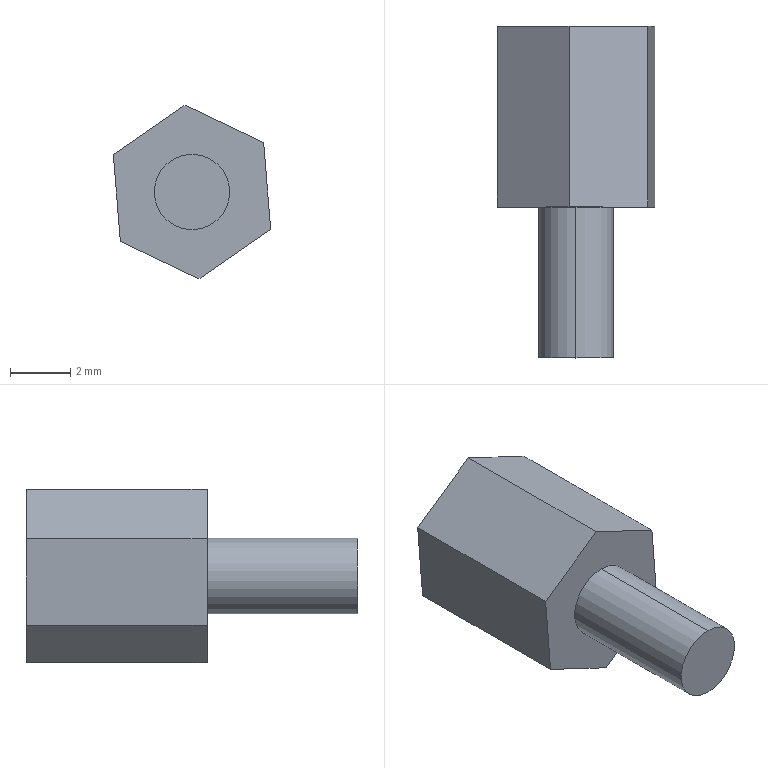Component | SolidWorks | Bolt-11 | 1 solid | 14 faces | box 5.22 x 11 x 5.75 mm | volume 130 mm3 | plane 10 | cylinder 4 | commonest cylinder face diameters 2.5 x4
build123d program:
from build123d import *

# Parameters (mm, degrees)
BOSS_EXTRUDE1_DEPTH = 6
SKETCH2_R           = 1.25
CUT_EXTRUDE1_DEPTH  = 5
SKETCH3_R           = 1.25
BOSS_EXTRUDE2_DEPTH = 5


with BuildPart() as part:
    # Sketch1 → Boss-Extrude1 (new body)
    with BuildSketch(Plane.XY):
        Polygon((2.877, 0.2318), (1.238, 2.608), (-1.639, 2.376), (-2.877, -0.2318), (-1.238, -2.608), (1.639, -2.376), align=None)
    extrude(amount=BOSS_EXTRUDE1_DEPTH)

    # Sketch2 → Cut-Extrude1 (cut)
    with BuildSketch(Plane(origin=(0, 0, 0), x_dir=(-1, 0, 0), z_dir=(0, 0, -1))):
        Circle(SKETCH2_R)
    extrude(amount=-CUT_EXTRUDE1_DEPTH, mode=Mode.SUBTRACT)

    # Sketch3 → Boss-Extrude2 (add)
    with BuildSketch(Plane.XY.offset(6)):
        with Locations(Location((0, 0, 0), (0, 0, 180))):
            Circle(SKETCH3_R)
    extrude(amount=BOSS_EXTRUDE2_DEPTH)


solid = part.part

# Placed as in the assembly
solid = solid.moved(Location((27.326, 19.961, 70.581), (90, 0, 90)))
STEP:
#1=COLOUR_RGB('',0.7922,0.8196,0.9333);
#2=FILL_AREA_STYLE_COLOUR('',#1);
#3=FILL_AREA_STYLE('',(#2));
#4=SURFACE_STYLE_FILL_AREA(#3);
#5=SURFACE_SIDE_STYLE('',(#4));
#6=SURFACE_STYLE_USAGE(.BOTH.,#5);
#7=PRESENTATION_STYLE_ASSIGNMENT((#6));
#8=CARTESIAN_POINT('',(1.076,0.3528,2.73));
#9=VERTEX_POINT('',#8);
#10=CARTESIAN_POINT('',(1.076,0.3528,2.828));
#11=VERTEX_POINT('',#10);
#12=CARTESIAN_POINT('',(1.076,0.3528,2.779));
#13=DIRECTION('',(-0.,-1.,-0.));
#14=DIRECTION('',(0.,0.,-1.));
#15=AXIS2_PLACEMENT_3D('',#12,#13,#14);
#16=CIRCLE('',#15,0.04921);
#17=EDGE_CURVE('',#9,#11,#16,.T.);
#18=ORIENTED_EDGE('',*,*,#17,.F.);
#19=CARTESIAN_POINT('',(1.076,0.5496,2.73));
#20=VERTEX_POINT('',#19);
#21=CARTESIAN_POINT('',(1.076,0.3528,2.73));
#22=DIRECTION('',(0.,1.,0.));
#23=VECTOR('',#22,39.37);
#24=LINE('',#21,#23);
#25=EDGE_CURVE('',#9,#20,#24,.T.);
#26=ORIENTED_EDGE('',*,*,#25,.T.);
#27=CARTESIAN_POINT('',(1.076,0.5496,2.828));
#28=VERTEX_POINT('',#27);
#29=CARTESIAN_POINT('',(1.076,0.5496,2.779));
#30=DIRECTION('',(-0.,-1.,-0.));
#31=DIRECTION('',(0.,0.,-1.));
#32=AXIS2_PLACEMENT_3D('',#29,#30,#31);
#33=CIRCLE('',#32,0.04921);
#34=EDGE_CURVE('',#20,#28,#33,.T.);
#35=ORIENTED_EDGE('',*,*,#34,.T.);
#36=CARTESIAN_POINT('',(1.076,0.3528,2.828));
#37=DIRECTION('',(0.,1.,0.));
#38=VECTOR('',#37,39.37);
#39=LINE('',#36,#38);
#40=EDGE_CURVE('',#11,#28,#39,.T.);
#41=ORIENTED_EDGE('',*,*,#40,.F.);
#42=EDGE_LOOP('',(#18,#26,#35,#41));
#43=FACE_OUTER_BOUND('',#42,.T.);
#44=CARTESIAN_POINT('',(1.076,0.3528,2.779));
#45=DIRECTION('',(0.,1.,0.));
#46=DIRECTION('',(-0.,-0.,1.));
#47=AXIS2_PLACEMENT_3D('',#44,#45,#46);
#48=CYLINDRICAL_SURFACE('',#47,0.04921);
#49=ADVANCED_FACE('',(#43),#48,.T.);
#50=CARTESIAN_POINT('',(1.076,0.589,2.73));
#51=VERTEX_POINT('',#50);
#52=CARTESIAN_POINT('',(1.076,0.589,2.828));
#53=VERTEX_POINT('',#52);
#54=CARTESIAN_POINT('',(1.076,0.589,2.779));
#55=DIRECTION('',(0.,1.,0.));
#56=DIRECTION('',(-0.,-0.,1.));
#57=AXIS2_PLACEMENT_3D('',#54,#55,#56);
#58=CIRCLE('',#57,0.04921);
#59=EDGE_CURVE('',#51,#53,#58,.T.);
#60=ORIENTED_EDGE('',*,*,#59,.F.);
#61=CARTESIAN_POINT('',(1.076,0.7859,2.73));
#62=VERTEX_POINT('',#61);
#63=CARTESIAN_POINT('',(1.076,0.589,2.73));
#64=DIRECTION('',(0.,1.,0.));
#65=VECTOR('',#64,39.37);
#66=LINE('',#63,#65);
#67=EDGE_CURVE('',#51,#62,#66,.T.);
#68=ORIENTED_EDGE('',*,*,#67,.T.);
#69=CARTESIAN_POINT('',(1.076,0.7859,2.828));
#70=VERTEX_POINT('',#69);
#71=CARTESIAN_POINT('',(1.076,0.7859,2.779));
#72=DIRECTION('',(0.,1.,0.));
#73=DIRECTION('',(-0.,-0.,1.));
#74=AXIS2_PLACEMENT_3D('',#71,#72,#73);
#75=CIRCLE('',#74,0.04921);
#76=EDGE_CURVE('',#62,#70,#75,.T.);
#77=ORIENTED_EDGE('',*,*,#76,.T.);
#78=CARTESIAN_POINT('',(1.076,0.589,2.828));
#79=DIRECTION('',(0.,1.,0.));
#80=VECTOR('',#79,39.37);
#81=LINE('',#78,#80);
#82=EDGE_CURVE('',#53,#70,#81,.T.);
#83=ORIENTED_EDGE('',*,*,#82,.F.);
#84=EDGE_LOOP('',(#60,#68,#77,#83));
#85=FACE_OUTER_BOUND('',#84,.T.);
#86=CARTESIAN_POINT('',(1.076,0.589,2.779));
#87=DIRECTION('',(0.,1.,0.));
#88=DIRECTION('',(-0.,-0.,1.));
#89=AXIS2_PLACEMENT_3D('',#86,#87,#88);
#90=CYLINDRICAL_SURFACE('',#89,0.04921);
#91=ADVANCED_FACE('',(#85),#90,.F.);
#92=CARTESIAN_POINT('',(0.9823,0.7859,2.714));
#93=VERTEX_POINT('',#92);
#94=CARTESIAN_POINT('',(1.085,0.7859,2.665));
#95=VERTEX_POINT('',#94);
#96=CARTESIAN_POINT('',(0.9823,0.7859,2.714));
#97=DIRECTION('',(0.9034,-0.,-0.4289));
#98=VECTOR('',#97,39.37);
#99=LINE('',#96,#98);
#100=EDGE_CURVE('',#93,#95,#99,.T.);
#101=ORIENTED_EDGE('',*,*,#100,.T.);
#102=CARTESIAN_POINT('',(1.085,0.5496,2.665));
#103=VERTEX_POINT('',#102);
#104=CARTESIAN_POINT('',(1.085,0.5496,2.665));
#105=DIRECTION('',(0.,1.,0.));
#106=VECTOR('',#105,39.37);
#107=LINE('',#104,#106);
#108=EDGE_CURVE('',#103,#95,#107,.T.);
#109=ORIENTED_EDGE('',*,*,#108,.F.);
#110=CARTESIAN_POINT('',(0.9823,0.5496,2.714));
#111=VERTEX_POINT('',#110);
#112=CARTESIAN_POINT('',(0.9823,0.5496,2.714));
#113=DIRECTION('',(0.9034,-0.,-0.4289));
#114=VECTOR('',#113,39.37);
#115=LINE('',#112,#114);
#116=EDGE_CURVE('',#111,#103,#115,.T.);
#117=ORIENTED_EDGE('',*,*,#116,.F.);
#118=CARTESIAN_POINT('',(0.9823,0.5496,2.714));
#119=DIRECTION('',(0.,1.,0.));
#120=VECTOR('',#119,39.37);
#121=LINE('',#118,#120);
#122=EDGE_CURVE('',#111,#93,#121,.T.);
#123=ORIENTED_EDGE('',*,*,#122,.T.);
#124=EDGE_LOOP('',(#101,#109,#117,#123));
#125=FACE_OUTER_BOUND('',#124,.T.);
#126=CARTESIAN_POINT('',(0.9823,0.5496,2.714));
#127=DIRECTION('',(0.4289,-0.,0.9034));
#128=DIRECTION('',(-0.9034,0.,0.4289));
#129=AXIS2_PLACEMENT_3D('',#126,#127,#128);
#130=PLANE('',#129);
#131=ADVANCED_FACE('',(#125),#130,.F.);
#132=CARTESIAN_POINT('',(1.179,0.7859,2.73));
#133=VERTEX_POINT('',#132);
#134=CARTESIAN_POINT('',(1.085,0.7859,2.665));
#135=DIRECTION('',(0.8231,-0.,0.5679));
#136=VECTOR('',#135,39.37);
#137=LINE('',#134,#136);
#138=EDGE_CURVE('',#95,#133,#137,.T.);
#139=ORIENTED_EDGE('',*,*,#138,.T.);
#140=CARTESIAN_POINT('',(1.179,0.5496,2.73));
#141=VERTEX_POINT('',#140);
#142=CARTESIAN_POINT('',(1.179,0.5496,2.73));
#143=DIRECTION('',(0.,1.,0.));
#144=VECTOR('',#143,39.37);
#145=LINE('',#142,#144);
#146=EDGE_CURVE('',#141,#133,#145,.T.);
#147=ORIENTED_EDGE('',*,*,#146,.F.);
#148=CARTESIAN_POINT('',(1.085,0.5496,2.665));
#149=DIRECTION('',(0.8231,-0.,0.5679));
#150=VECTOR('',#149,39.37);
#151=LINE('',#148,#150);
#152=EDGE_CURVE('',#103,#141,#151,.T.);
#153=ORIENTED_EDGE('',*,*,#152,.F.);
#154=ORIENTED_EDGE('',*,*,#108,.T.);
#155=EDGE_LOOP('',(#139,#147,#153,#154));
#156=FACE_OUTER_BOUND('',#155,.T.);
#157=CARTESIAN_POINT('',(1.085,0.5496,2.665));
#158=DIRECTION('',(-0.5679,-0.,0.8231));
#159=DIRECTION('',(-0.8231,0.,-0.5679));
#160=AXIS2_PLACEMENT_3D('',#157,#158,#159);
#161=PLANE('',#160);
#162=ADVANCED_FACE('',(#156),#161,.F.);
#163=CARTESIAN_POINT('',(1.169,0.7859,2.843));
#164=VERTEX_POINT('',#163);
#165=CARTESIAN_POINT('',(1.179,0.7859,2.73));
#166=DIRECTION('',(-0.08029,-0.,0.9968));
#167=VECTOR('',#166,39.37);
#168=LINE('',#165,#167);
#169=EDGE_CURVE('',#133,#164,#168,.T.);
#170=ORIENTED_EDGE('',*,*,#169,.T.);
#171=CARTESIAN_POINT('',(1.169,0.5496,2.843));
#172=VERTEX_POINT('',#171);
#173=CARTESIAN_POINT('',(1.169,0.5496,2.843));
#174=DIRECTION('',(0.,1.,0.));
#175=VECTOR('',#174,39.37);
#176=LINE('',#173,#175);
#177=EDGE_CURVE('',#172,#164,#176,.T.);
#178=ORIENTED_EDGE('',*,*,#177,.F.);
#179=CARTESIAN_POINT('',(1.179,0.5496,2.73));
#180=DIRECTION('',(-0.08029,-0.,0.9968));
#181=VECTOR('',#180,39.37);
#182=LINE('',#179,#181);
#183=EDGE_CURVE('',#141,#172,#182,.T.);
#184=ORIENTED_EDGE('',*,*,#183,.F.);
#185=ORIENTED_EDGE('',*,*,#146,.T.);
#186=EDGE_LOOP('',(#170,#178,#184,#185));
#187=FACE_OUTER_BOUND('',#186,.T.);
#188=CARTESIAN_POINT('',(1.179,0.5496,2.73));
#189=DIRECTION('',(-0.9968,0.,-0.08029));
#190=DIRECTION('',(0.08029,0.,-0.9968));
#191=AXIS2_PLACEMENT_3D('',#188,#189,#190);
#192=PLANE('',#191);
#193=ADVANCED_FACE('',(#187),#192,.F.);
#194=CARTESIAN_POINT('',(1.067,0.7859,2.892));
#195=VERTEX_POINT('',#194);
#196=CARTESIAN_POINT('',(1.169,0.7859,2.843));
#197=DIRECTION('',(-0.9034,0.,0.4289));
#198=VECTOR('',#197,39.37);
#199=LINE('',#196,#198);
#200=EDGE_CURVE('',#164,#195,#199,.T.);
#201=ORIENTED_EDGE('',*,*,#200,.T.);
#202=CARTESIAN_POINT('',(1.067,0.5496,2.892));
#203=VERTEX_POINT('',#202);
#204=CARTESIAN_POINT('',(1.067,0.5496,2.892));
#205=DIRECTION('',(0.,1.,0.));
#206=VECTOR('',#205,39.37);
#207=LINE('',#204,#206);
#208=EDGE_CURVE('',#203,#195,#207,.T.);
#209=ORIENTED_EDGE('',*,*,#208,.F.);
#210=CARTESIAN_POINT('',(1.169,0.5496,2.843));
#211=DIRECTION('',(-0.9034,0.,0.4289));
#212=VECTOR('',#211,39.37);
#213=LINE('',#210,#212);
#214=EDGE_CURVE('',#172,#203,#213,.T.);
#215=ORIENTED_EDGE('',*,*,#214,.F.);
#216=ORIENTED_EDGE('',*,*,#177,.T.);
#217=EDGE_LOOP('',(#201,#209,#215,#216));
#218=FACE_OUTER_BOUND('',#217,.T.);
#219=CARTESIAN_POINT('',(1.169,0.5496,2.843));
#220=DIRECTION('',(-0.4289,0.,-0.9034));
#221=DIRECTION('',(0.9034,-0.,-0.4289));
#222=AXIS2_PLACEMENT_3D('',#219,#220,#221);
#223=PLANE('',#222);
#224=ADVANCED_FACE('',(#218),#223,.F.);
#225=CARTESIAN_POINT('',(0.9732,0.7859,2.828));
#226=VERTEX_POINT('',#225);
#227=CARTESIAN_POINT('',(1.067,0.7859,2.892));
#228=DIRECTION('',(-0.8231,0.,-0.5679));
#229=VECTOR('',#228,39.37);
#230=LINE('',#227,#229);
#231=EDGE_CURVE('',#195,#226,#230,.T.);
#232=ORIENTED_EDGE('',*,*,#231,.T.);
#233=CARTESIAN_POINT('',(0.9732,0.5496,2.828));
#234=VERTEX_POINT('',#233);
#235=CARTESIAN_POINT('',(0.9732,0.5496,2.828));
#236=DIRECTION('',(0.,1.,0.));
#237=VECTOR('',#236,39.37);
#238=LINE('',#235,#237);
#239=EDGE_CURVE('',#234,#226,#238,.T.);
#240=ORIENTED_EDGE('',*,*,#239,.F.);
#241=CARTESIAN_POINT('',(1.067,0.5496,2.892));
#242=DIRECTION('',(-0.8231,0.,-0.5679));
#243=VECTOR('',#242,39.37);
#244=LINE('',#241,#243);
#245=EDGE_CURVE('',#203,#234,#244,.T.);
#246=ORIENTED_EDGE('',*,*,#245,.F.);
#247=ORIENTED_EDGE('',*,*,#208,.T.);
#248=EDGE_LOOP('',(#232,#240,#246,#247));
#249=FACE_OUTER_BOUND('',#248,.T.);
#250=CARTESIAN_POINT('',(1.067,0.5496,2.892));
#251=DIRECTION('',(0.5679,0.,-0.8231));
#252=DIRECTION('',(0.8231,-0.,0.5679));
#253=AXIS2_PLACEMENT_3D('',#250,#251,#252);
#254=PLANE('',#253);
#255=ADVANCED_FACE('',(#249),#254,.F.);
#256=CARTESIAN_POINT('',(0.9732,0.7859,2.828));
#257=DIRECTION('',(0.08029,0.,-0.9968));
#258=VECTOR('',#257,39.37);
#259=LINE('',#256,#258);
#260=EDGE_CURVE('',#226,#93,#259,.T.);
#261=ORIENTED_EDGE('',*,*,#260,.T.);
#262=ORIENTED_EDGE('',*,*,#122,.F.);
#263=CARTESIAN_POINT('',(0.9732,0.5496,2.828));
#264=DIRECTION('',(0.08029,0.,-0.9968));
#265=VECTOR('',#264,39.37);
#266=LINE('',#263,#265);
#267=EDGE_CURVE('',#234,#111,#266,.T.);
#268=ORIENTED_EDGE('',*,*,#267,.F.);
#269=ORIENTED_EDGE('',*,*,#239,.T.);
#270=EDGE_LOOP('',(#261,#262,#268,#269));
#271=FACE_OUTER_BOUND('',#270,.T.);
#272=CARTESIAN_POINT('',(0.9732,0.5496,2.828));
#273=DIRECTION('',(0.9968,-0.,0.08029));
#274=DIRECTION('',(-0.08029,-0.,0.9968));
#275=AXIS2_PLACEMENT_3D('',#272,#273,#274);
#276=PLANE('',#275);
#277=ADVANCED_FACE('',(#271),#276,.F.);
#278=CARTESIAN_POINT('',(1.076,0.5496,2.779));
#279=DIRECTION('',(-0.,-1.,-0.));
#280=DIRECTION('',(0.,0.,-1.));
#281=AXIS2_PLACEMENT_3D('',#278,#279,#280);
#282=CIRCLE('',#281,0.04921);
#283=EDGE_CURVE('',#28,#20,#282,.T.);
#284=ORIENTED_EDGE('',*,*,#283,.F.);
#285=ORIENTED_EDGE('',*,*,#34,.F.);
#286=EDGE_LOOP('',(#284,#285));
#287=FACE_BOUND('',#286,.T.);
#288=ORIENTED_EDGE('',*,*,#116,.T.);
#289=ORIENTED_EDGE('',*,*,#152,.T.);
#290=ORIENTED_EDGE('',*,*,#183,.T.);
#291=ORIENTED_EDGE('',*,*,#214,.T.);
#292=ORIENTED_EDGE('',*,*,#245,.T.);
#293=ORIENTED_EDGE('',*,*,#267,.T.);
#294=EDGE_LOOP('',(#288,#289,#290,#291,#292,#293));
#295=FACE_OUTER_BOUND('',#294,.T.);
#296=CARTESIAN_POINT('',(1.076,0.5496,2.779));
#297=DIRECTION('',(-0.,-1.,-0.));
#298=DIRECTION('',(0.,0.,-1.));
#299=AXIS2_PLACEMENT_3D('',#296,#297,#298);
#300=PLANE('',#299);
#301=ADVANCED_FACE('',(#287,#295),#300,.T.);
#302=CARTESIAN_POINT('',(1.076,0.7859,2.779));
#303=DIRECTION('',(0.,1.,0.));
#304=DIRECTION('',(-0.,-0.,1.));
#305=AXIS2_PLACEMENT_3D('',#302,#303,#304);
#306=CIRCLE('',#305,0.04921);
#307=EDGE_CURVE('',#70,#62,#306,.T.);
#308=ORIENTED_EDGE('',*,*,#307,.F.);
#309=ORIENTED_EDGE('',*,*,#76,.F.);
#310=EDGE_LOOP('',(#308,#309));
#311=FACE_BOUND('',#310,.T.);
#312=ORIENTED_EDGE('',*,*,#100,.F.);
#313=ORIENTED_EDGE('',*,*,#260,.F.);
#314=ORIENTED_EDGE('',*,*,#231,.F.);
#315=ORIENTED_EDGE('',*,*,#200,.F.);
#316=ORIENTED_EDGE('',*,*,#169,.F.);
#317=ORIENTED_EDGE('',*,*,#138,.F.);
#318=EDGE_LOOP('',(#312,#313,#314,#315,#316,#317));
#319=FACE_OUTER_BOUND('',#318,.T.);
#320=CARTESIAN_POINT('',(1.076,0.7859,2.779));
#321=DIRECTION('',(-0.,-1.,-0.));
#322=DIRECTION('',(0.,0.,-1.));
#323=AXIS2_PLACEMENT_3D('',#320,#321,#322);
#324=PLANE('',#323);
#325=ADVANCED_FACE('',(#311,#319),#324,.F.);
#326=ORIENTED_EDGE('',*,*,#67,.F.);
#327=CARTESIAN_POINT('',(1.076,0.589,2.779));
#328=DIRECTION('',(0.,1.,0.));
#329=DIRECTION('',(-0.,-0.,1.));
#330=AXIS2_PLACEMENT_3D('',#327,#328,#329);
#331=CIRCLE('',#330,0.04921);
#332=EDGE_CURVE('',#53,#51,#331,.T.);
#333=ORIENTED_EDGE('',*,*,#332,.F.);
#334=ORIENTED_EDGE('',*,*,#82,.T.);
#335=ORIENTED_EDGE('',*,*,#307,.T.);
#336=EDGE_LOOP('',(#326,#333,#334,#335));
#337=FACE_OUTER_BOUND('',#336,.T.);
#338=CARTESIAN_POINT('',(1.076,0.589,2.779));
#339=DIRECTION('',(0.,1.,0.));
#340=DIRECTION('',(-0.,-0.,1.));
#341=AXIS2_PLACEMENT_3D('',#338,#339,#340);
#342=CYLINDRICAL_SURFACE('',#341,0.04921);
#343=ADVANCED_FACE('',(#337),#342,.F.);
#344=ORIENTED_EDGE('',*,*,#332,.T.);
#345=ORIENTED_EDGE('',*,*,#59,.T.);
#346=EDGE_LOOP('',(#344,#345));
#347=FACE_OUTER_BOUND('',#346,.T.);
#348=CARTESIAN_POINT('',(1.076,0.589,2.779));
#349=DIRECTION('',(0.,1.,0.));
#350=DIRECTION('',(-0.,-0.,1.));
#351=AXIS2_PLACEMENT_3D('',#348,#349,#350);
#352=PLANE('',#351);
#353=ADVANCED_FACE('',(#347),#352,.T.);
#354=ORIENTED_EDGE('',*,*,#25,.F.);
#355=CARTESIAN_POINT('',(1.076,0.3528,2.779));
#356=DIRECTION('',(-0.,-1.,-0.));
#357=DIRECTION('',(0.,0.,-1.));
#358=AXIS2_PLACEMENT_3D('',#355,#356,#357);
#359=CIRCLE('',#358,0.04921);
#360=EDGE_CURVE('',#11,#9,#359,.T.);
#361=ORIENTED_EDGE('',*,*,#360,.F.);
#362=ORIENTED_EDGE('',*,*,#40,.T.);
#363=ORIENTED_EDGE('',*,*,#283,.T.);
#364=EDGE_LOOP('',(#354,#361,#362,#363));
#365=FACE_OUTER_BOUND('',#364,.T.);
#366=CARTESIAN_POINT('',(1.076,0.3528,2.779));
#367=DIRECTION('',(0.,1.,0.));
#368=DIRECTION('',(-0.,-0.,1.));
#369=AXIS2_PLACEMENT_3D('',#366,#367,#368);
#370=CYLINDRICAL_SURFACE('',#369,0.04921);
#371=ADVANCED_FACE('',(#365),#370,.T.);
#372=ORIENTED_EDGE('',*,*,#360,.T.);
#373=ORIENTED_EDGE('',*,*,#17,.T.);
#374=EDGE_LOOP('',(#372,#373));
#375=FACE_OUTER_BOUND('',#374,.T.);
#376=CARTESIAN_POINT('',(1.076,0.3528,2.779));
#377=DIRECTION('',(-0.,-1.,-0.));
#378=DIRECTION('',(0.,0.,-1.));
#379=AXIS2_PLACEMENT_3D('',#376,#377,#378);
#380=PLANE('',#379);
#381=ADVANCED_FACE('',(#375),#380,.T.);
#382=CLOSED_SHELL('',(#49,#91,#131,#162,#193,#224,#255,#277,#301,#325,#343,#353,#371,#381));
#383=MANIFOLD_SOLID_BREP('',#382);
#384=STYLED_ITEM('',(#7),#383);
#385=(LENGTH_UNIT()NAMED_UNIT(*)SI_UNIT($,.METRE.));
#386=LENGTH_MEASURE_WITH_UNIT(LENGTH_MEASURE(0.0254),#385);
#387=DIMENSIONAL_EXPONENTS(1.,0.,0.,0.,0.,0.,0.);
#388=(CONVERSION_BASED_UNIT('',#386)LENGTH_UNIT()NAMED_UNIT(#387));
#389=UNCERTAINTY_MEASURE_WITH_UNIT(LENGTH_MEASURE(0.00001),#388,'','');
#390=(NAMED_UNIT(*)PLANE_ANGLE_UNIT()SI_UNIT($,.RADIAN.));
#391=(NAMED_UNIT(*)SI_UNIT($,.STERADIAN.)SOLID_ANGLE_UNIT());
#392=(GEOMETRIC_REPRESENTATION_CONTEXT(3)GLOBAL_UNCERTAINTY_ASSIGNED_CONTEXT((#389))GLOBAL_UNIT_ASSIGNED_CONTEXT((#388,#390,#391))REPRESENTATION_CONTEXT('',''));
#393=MECHANICAL_DESIGN_GEOMETRIC_PRESENTATION_REPRESENTATION('',(#384),#392);
#394=PRESENTATION_LAYER_ASSIGNMENT('','',(#384));
#395=CARTESIAN_POINT('',(0.,0.,0.));
#396=DIRECTION('',(0.,0.,1.));
#397=DIRECTION('',(1.,0.,0.));
#398=AXIS2_PLACEMENT_3D('',#395,#396,#397);
#399=(LENGTH_UNIT()NAMED_UNIT(*)SI_UNIT($,.METRE.));
#400=LENGTH_MEASURE_WITH_UNIT(LENGTH_MEASURE(0.0254),#399);
#401=DIMENSIONAL_EXPONENTS(1.,0.,0.,0.,0.,0.,0.);
#402=(CONVERSION_BASED_UNIT('',#400)LENGTH_UNIT()NAMED_UNIT(#401));
#403=UNCERTAINTY_MEASURE_WITH_UNIT(LENGTH_MEASURE(0.00001),#402,'','');
#404=(NAMED_UNIT(*)PLANE_ANGLE_UNIT()SI_UNIT($,.RADIAN.));
#405=(NAMED_UNIT(*)SI_UNIT($,.STERADIAN.)SOLID_ANGLE_UNIT());
#406=(GEOMETRIC_REPRESENTATION_CONTEXT(3)GLOBAL_UNCERTAINTY_ASSIGNED_CONTEXT((#403))GLOBAL_UNIT_ASSIGNED_CONTEXT((#402,#404,#405))REPRESENTATION_CONTEXT('',''));
#407=ADVANCED_BREP_SHAPE_REPRESENTATION('',(#383,#398),#406);